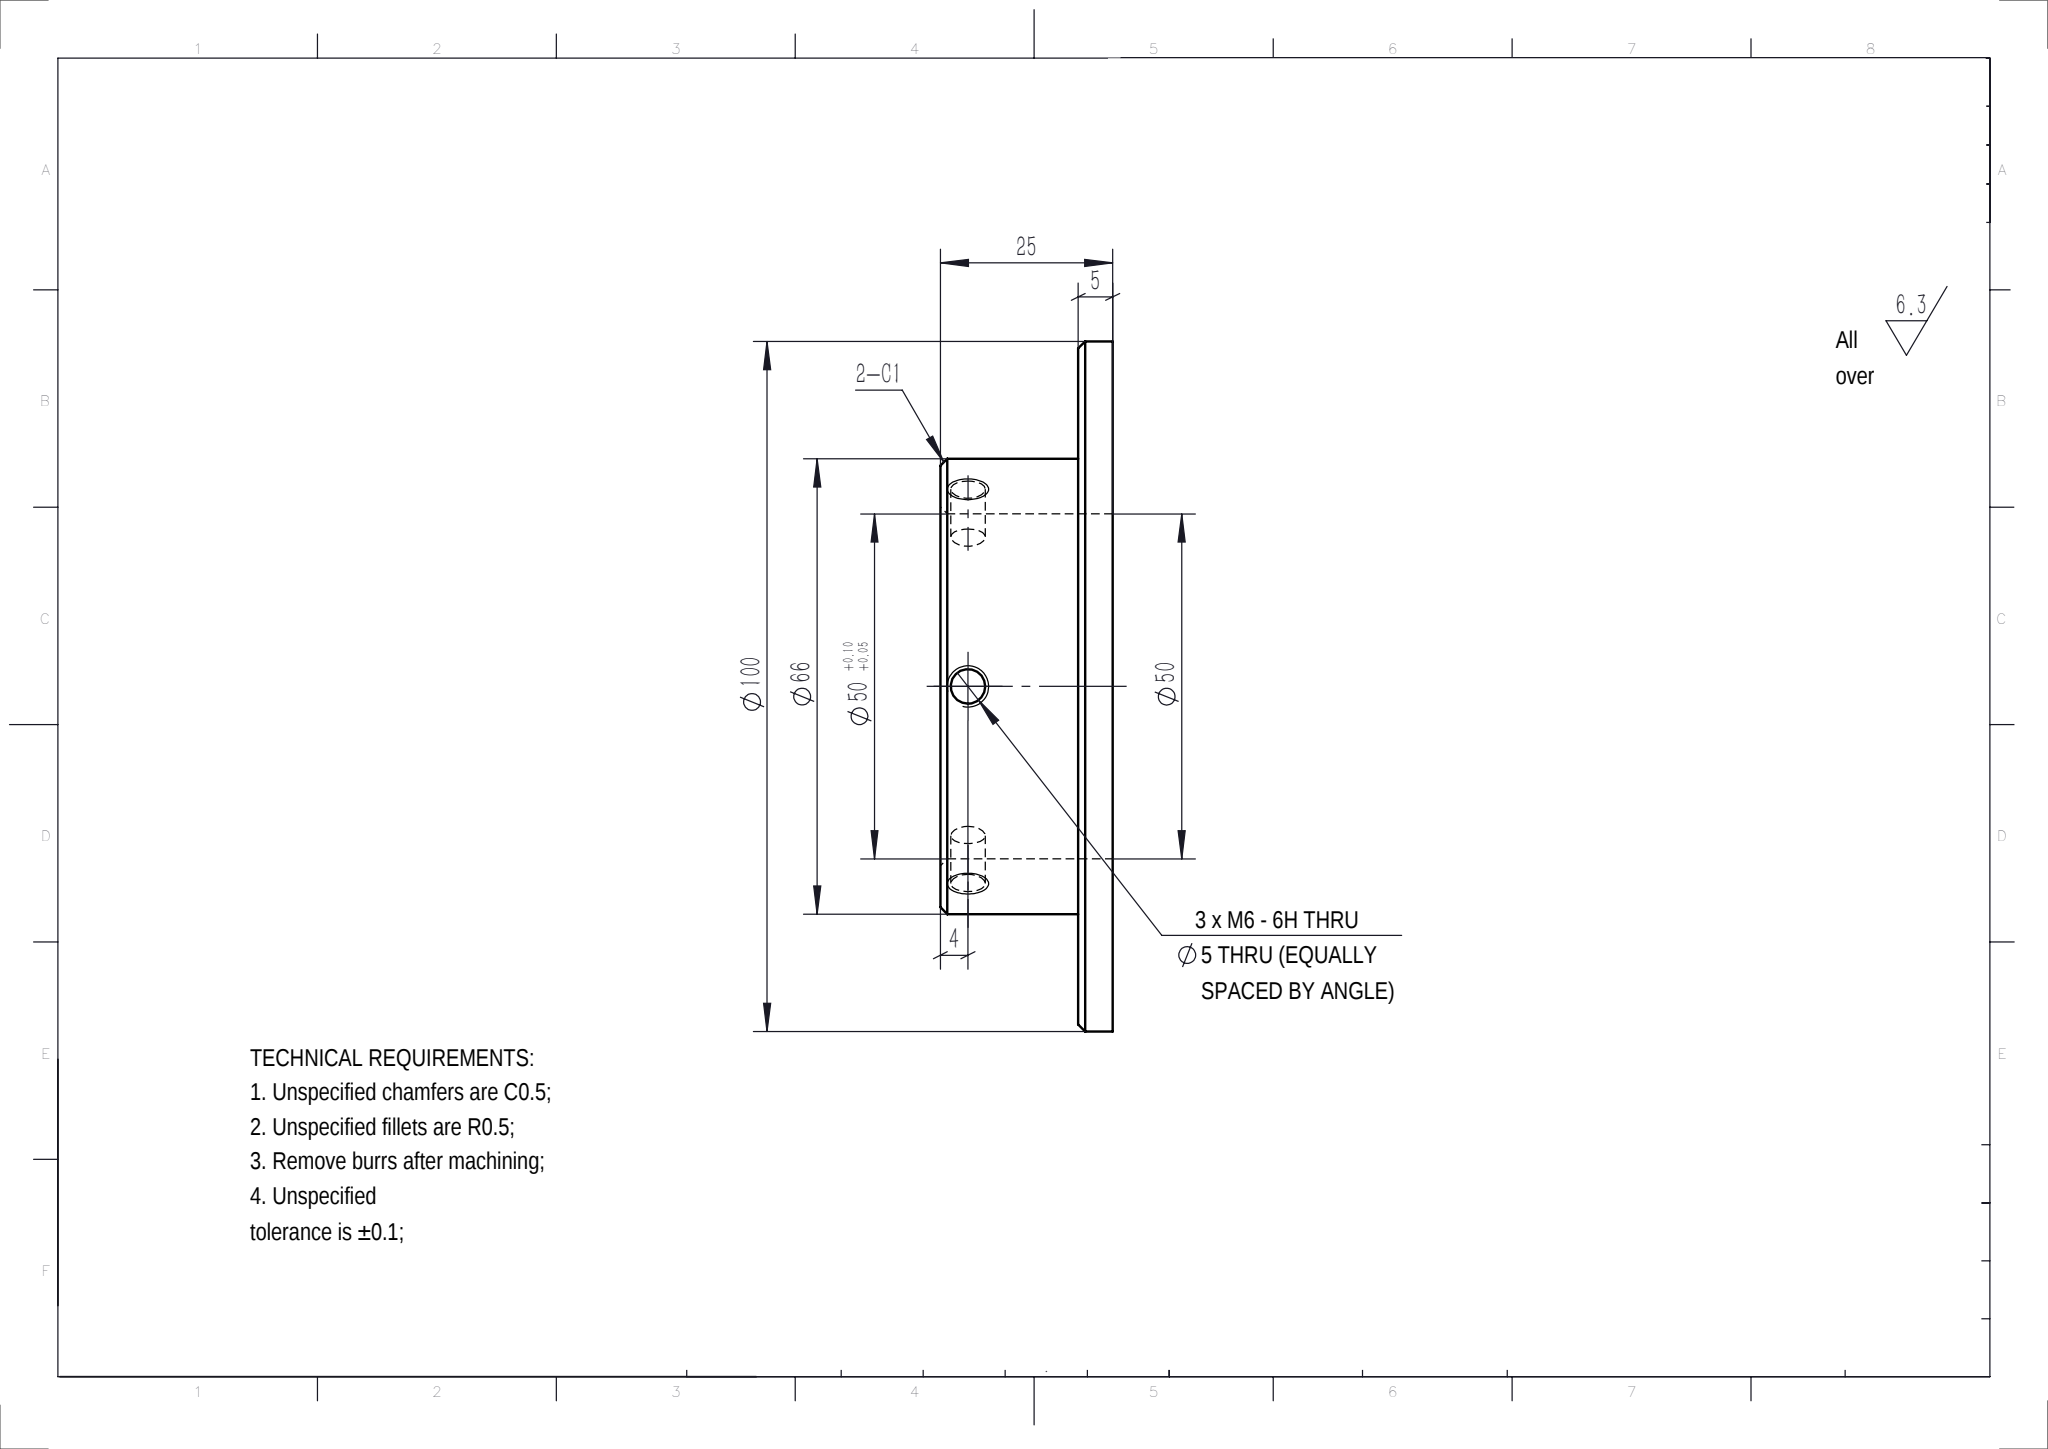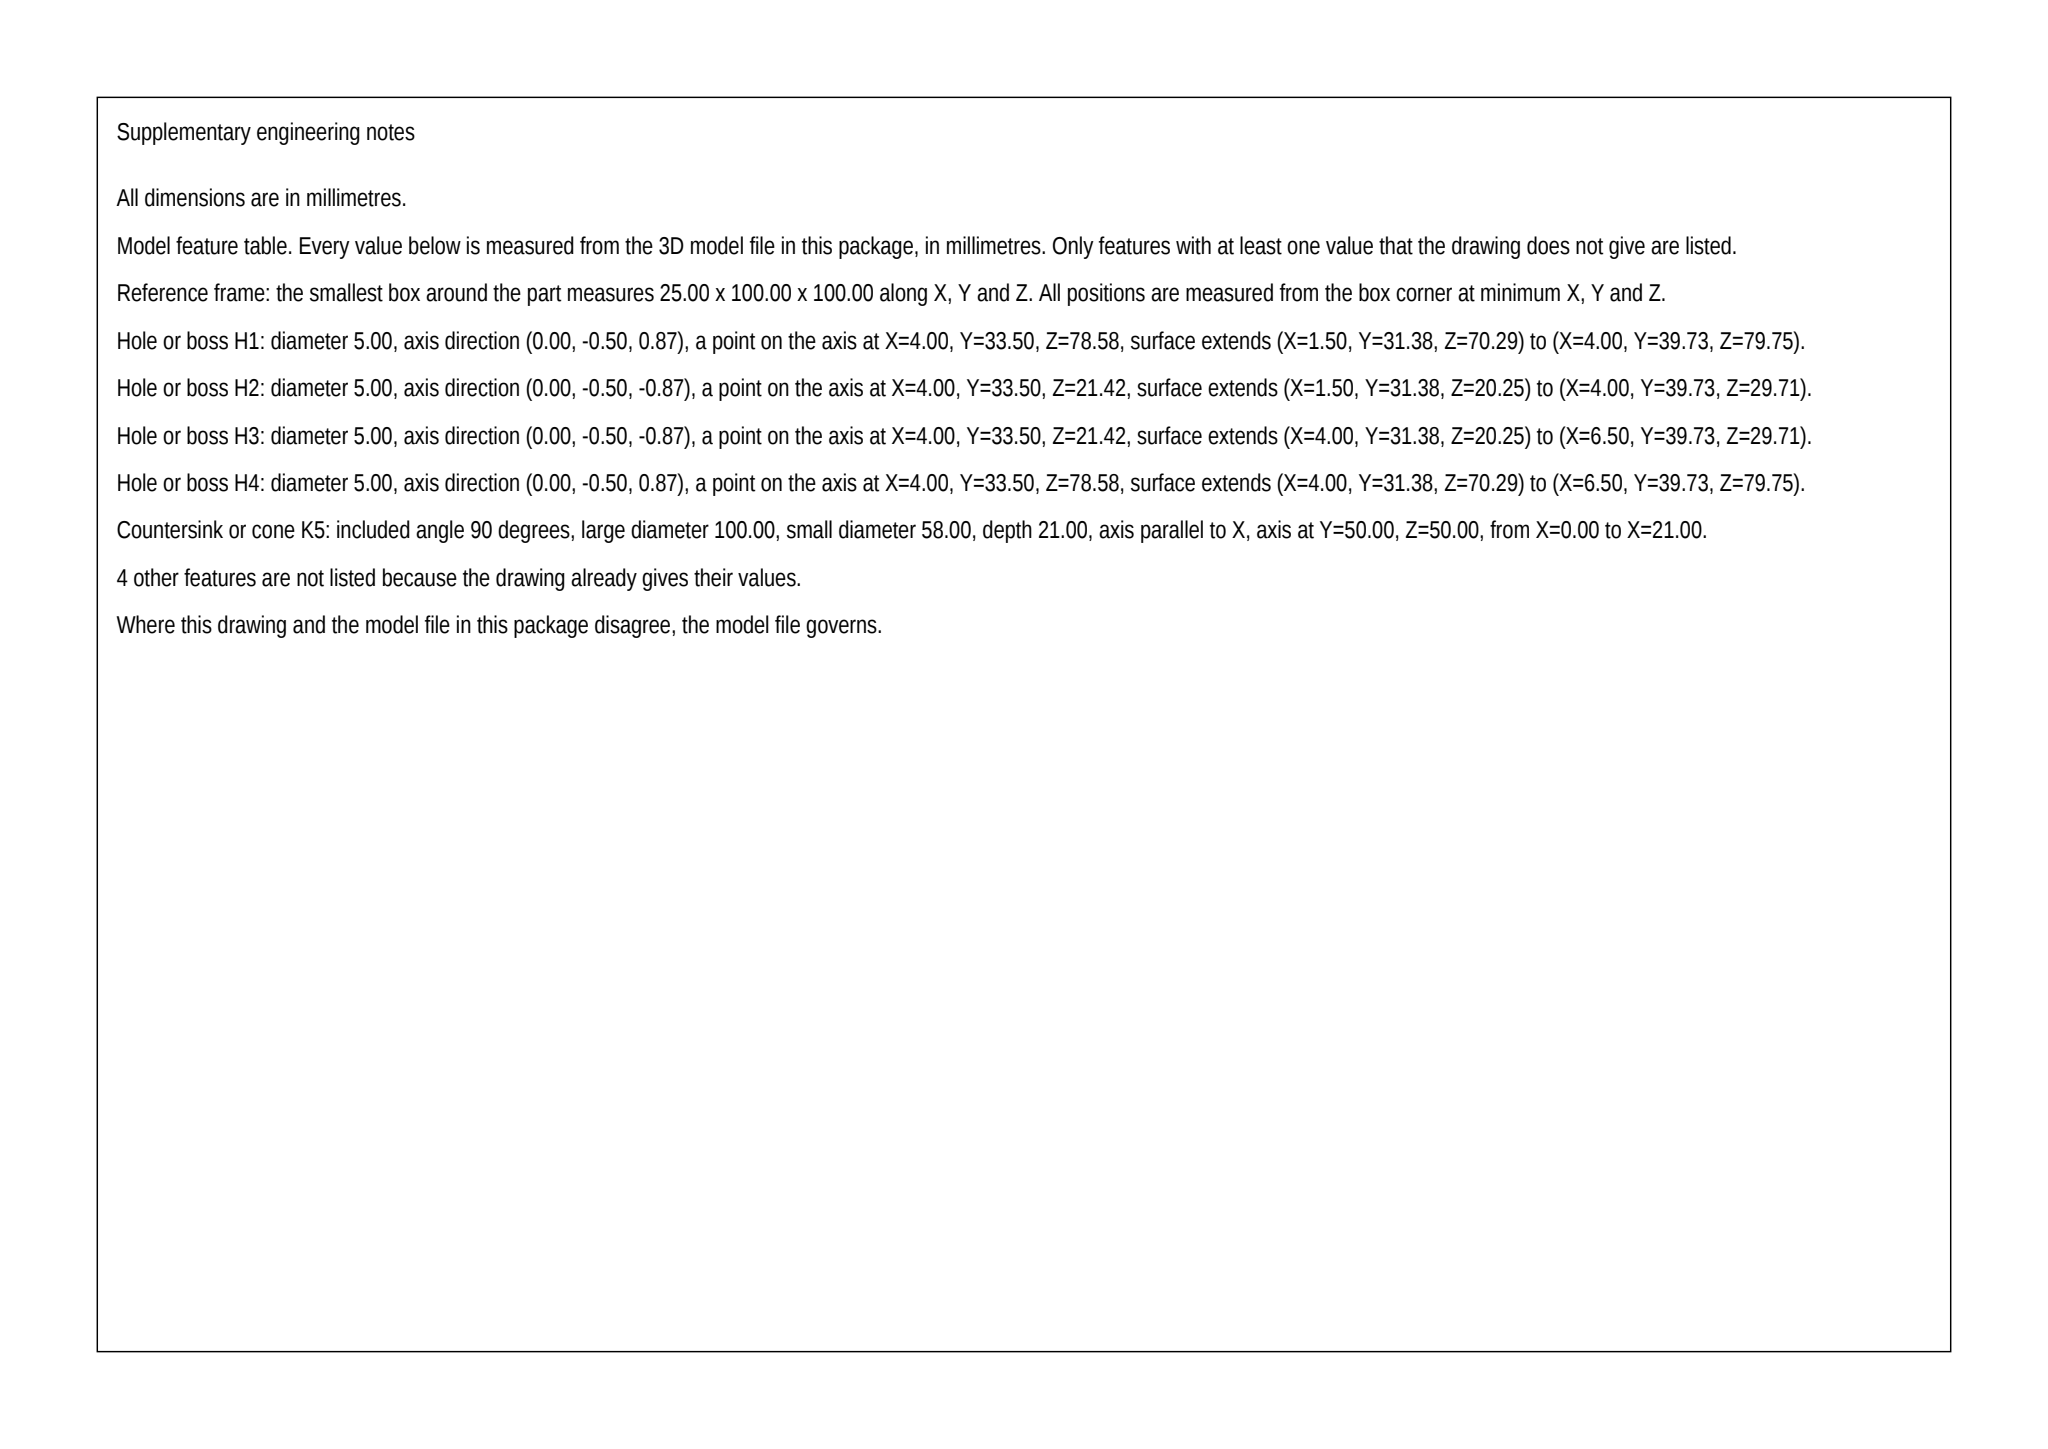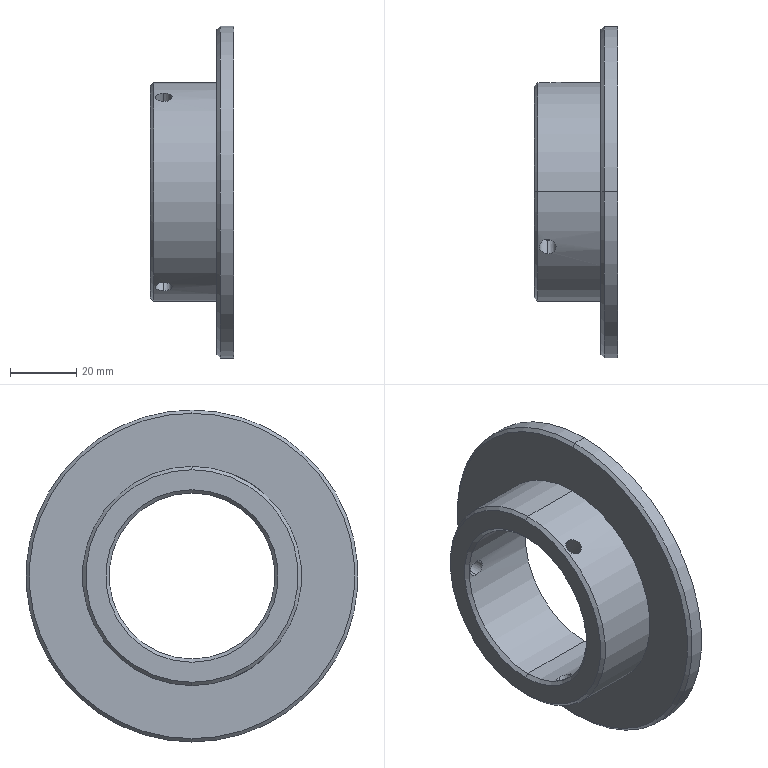Part | SolidWorks | mm | 1 solid | 21 faces | box 25 x 100 x 100 mm | volume 57796 mm3 | cylinder 12 | cone 6 | plane 3 | commonest cylinder face diameters 5 x6 66 x2 50 x2 100 x2
build123d program:
from build123d import *

# Parameters (mm, degrees)
M6_TAPPED_HOLE1_REACH  = 101.146
M6_TAPPED_HOLE1_BORE_R = 2.5
CIRPATTERN1_COUNT      = 3
CHAMFER1_SIZE          = 1


with BuildPart() as part:
    # Sketch1 → Revolve1 (revolve)
    with BuildSketch(Plane.XY, mode=Mode.PRIVATE) as revolve1_sk:
        Polygon((0, 33), (0, 50), (5, 50), (5, 25), (-20, 25), (-20, 33), align=None)
    revolve(revolve1_sk.sketch.rotate(Axis((0, 0, 0), (1, 0, 0)), 90), axis=Axis((0, 0, 0), (1, 0, 0)))

    # M6 Tapped Hole1 bore (on position points) → M6 Tapped Hole1 (cut, up to next)
    with BuildSketch(Plane(origin=(-16, 33, 0), x_dir=(0, 0, 1), z_dir=(0, 1, 0)), mode=Mode.PRIVATE) as m6_tapped_hole1_sk1:
        Circle(M6_TAPPED_HOLE1_BORE_R)
    m6_tapped_hole1_tool1 = extrude(m6_tapped_hole1_sk1.sketch, amount=-M6_TAPPED_HOLE1_REACH, mode=Mode.PRIVATE) & part.part
    m6_tapped_hole1 = m6_tapped_hole1_tool1.solids().sort_by_distance((-16, 33, 0))[0]
    add(m6_tapped_hole1, mode=Mode.SUBTRACT)

    # CirPattern1: M6 Tapped Hole1 ×3 about axis
    cirpattern1_axis = Axis((-20, 0, 0), (-1, 0, 0))
    for i in range(1, CIRPATTERN1_COUNT):
        add(m6_tapped_hole1.rotate(cirpattern1_axis, i * 360 / CIRPATTERN1_COUNT), mode=Mode.SUBTRACT)

    # Chamfer1
    chamfer1_edges = [part.edges().sort_by_distance(p)[0] for p in [
        (0, 0, -50),
        (-20, 0, -33),
        (-20, 0, -25),
    ]]
    chamfer(chamfer1_edges, length=CHAMFER1_SIZE)


solid = part.part